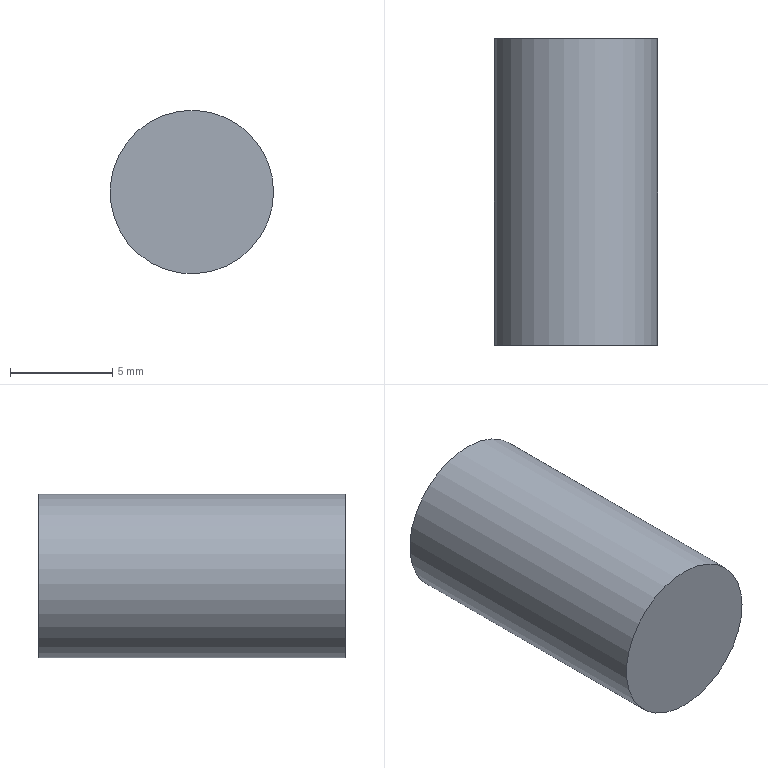Component | NX | 11_SMALL_PISTON | 1 solid | 3 faces | box 8 x 15 x 8 mm | volume 754 mm3 | plane 2 | cylinder 1 | commonest cylinder face diameters 8 x1
STEP:
#1=CARTESIAN_POINT('',(0.,0.,0.));
#2=DIRECTION('',(0.,0.,1.));
#3=DIRECTION('',(1.,0.,0.));
#4=AXIS2_PLACEMENT_3D('',#1,#2,#3);
#5=CARTESIAN_POINT('',(-55.735,168.794,-236.031));
#6=VERTEX_POINT('',#5);
#7=CARTESIAN_POINT('',(-59.084,168.794,-238.219));
#8=DIRECTION('',(0.,-1.,0.));
#9=DIRECTION('',(0.8372,0.,0.5469));
#10=AXIS2_PLACEMENT_3D('',#7,#8,#9);
#11=CIRCLE('',#10,4.);
#12=CARTESIAN_POINT('',(-59.084,168.794,-238.219));
#13=DIRECTION('',(0.,1.,0.));
#14=DIRECTION('',(0.8372,0.,0.5469));
#15=AXIS2_PLACEMENT_3D('',#12,#13,#14);
#16=PLANE('',#15);
#17=CARTESIAN_POINT('',(4.,-0.));
#18=CARTESIAN_POINT('',(4.,-6.928));
#19=CARTESIAN_POINT('',(-2.,-3.464));
#20=CARTESIAN_POINT('',(-8.,0.));
#21=CARTESIAN_POINT('',(-2.,3.464));
#22=CARTESIAN_POINT('',(4.,6.928));
#23=CARTESIAN_POINT('',(4.,-0.));
#24=(BOUNDED_CURVE()B_SPLINE_CURVE(2,(#17,#18,#19,#20,#21,#22,#23),.UNSPECIFIED.,.T.,.F.)B_SPLINE_CURVE_WITH_KNOTS((1,2,2,2,2,1),(-2.094,0.,2.094,4.189,6.283,8.378),.UNSPECIFIED.)CURVE()GEOMETRIC_REPRESENTATION_ITEM()RATIONAL_B_SPLINE_CURVE((1.,0.5,1.,0.5,1.,0.5,1.))REPRESENTATION_ITEM(''));
#25=(GEOMETRIC_REPRESENTATION_CONTEXT(2)PARAMETRIC_REPRESENTATION_CONTEXT()REPRESENTATION_CONTEXT('',''));
#26=DEFINITIONAL_REPRESENTATION('',(#24),#25);
#27=PCURVE('',#16,#26);
#28=CARTESIAN_POINT('',(-59.084,153.794,-238.219));
#29=DIRECTION('',(0.,1.,0.));
#30=DIRECTION('',(0.8372,0.,0.5469));
#31=AXIS2_PLACEMENT_3D('',#28,#29,#30);
#32=CYLINDRICAL_SURFACE('',#31,4.);
#33=CARTESIAN_POINT('',(6.283,15.));
#34=DIRECTION('',(-1.,0.));
#35=VECTOR('',#34,1.);
#36=LINE('',#33,#35);
#37=(GEOMETRIC_REPRESENTATION_CONTEXT(2)PARAMETRIC_REPRESENTATION_CONTEXT()REPRESENTATION_CONTEXT('',''));
#38=DEFINITIONAL_REPRESENTATION('',(#36),#37);
#39=PCURVE('',#32,#38);
#40=SURFACE_CURVE('',#11,(#27,#39),.PCURVE_S1.);
#41=EDGE_CURVE('',#6,#6,#40,.T.);
#42=ORIENTED_EDGE('',*,*,#41,.F.);
#43=EDGE_LOOP('',(#42));
#44=FACE_BOUND('',#43,.T.);
#45=ADVANCED_FACE('',(#44),#16,.T.);
#46=CARTESIAN_POINT('',(-55.735,153.794,-236.031));
#47=VERTEX_POINT('',#46);
#48=CARTESIAN_POINT('',(-59.084,153.794,-238.219));
#49=DIRECTION('',(0.,1.,0.));
#50=DIRECTION('',(0.8372,0.,0.5469));
#51=AXIS2_PLACEMENT_3D('',#48,#49,#50);
#52=CIRCLE('',#51,4.);
#53=CARTESIAN_POINT('',(-59.084,153.794,-238.219));
#54=DIRECTION('',(0.,-1.,0.));
#55=DIRECTION('',(-0.8372,0.,-0.5469));
#56=AXIS2_PLACEMENT_3D('',#53,#54,#55);
#57=PLANE('',#56);
#58=CARTESIAN_POINT('',(-4.,-0.));
#59=CARTESIAN_POINT('',(-4.,6.928));
#60=CARTESIAN_POINT('',(2.,3.464));
#61=CARTESIAN_POINT('',(8.,0.));
#62=CARTESIAN_POINT('',(2.,-3.464));
#63=CARTESIAN_POINT('',(-4.,-6.928));
#64=CARTESIAN_POINT('',(-4.,-0.));
#65=(BOUNDED_CURVE()B_SPLINE_CURVE(2,(#58,#59,#60,#61,#62,#63,#64),.UNSPECIFIED.,.T.,.F.)B_SPLINE_CURVE_WITH_KNOTS((1,2,2,2,2,1),(-2.094,0.,2.094,4.189,6.283,8.378),.UNSPECIFIED.)CURVE()GEOMETRIC_REPRESENTATION_ITEM()RATIONAL_B_SPLINE_CURVE((1.,0.5,1.,0.5,1.,0.5,1.))REPRESENTATION_ITEM(''));
#66=(GEOMETRIC_REPRESENTATION_CONTEXT(2)PARAMETRIC_REPRESENTATION_CONTEXT()REPRESENTATION_CONTEXT('',''));
#67=DEFINITIONAL_REPRESENTATION('',(#65),#66);
#68=PCURVE('',#57,#67);
#69=CARTESIAN_POINT('',(0.,0.));
#70=DIRECTION('',(1.,0.));
#71=VECTOR('',#70,1.);
#72=LINE('',#69,#71);
#73=(GEOMETRIC_REPRESENTATION_CONTEXT(2)PARAMETRIC_REPRESENTATION_CONTEXT()REPRESENTATION_CONTEXT('',''));
#74=DEFINITIONAL_REPRESENTATION('',(#72),#73);
#75=PCURVE('',#32,#74);
#76=SURFACE_CURVE('',#52,(#68,#75),.PCURVE_S1.);
#77=EDGE_CURVE('',#47,#47,#76,.T.);
#78=ORIENTED_EDGE('',*,*,#77,.F.);
#79=EDGE_LOOP('',(#78));
#80=FACE_BOUND('',#79,.T.);
#81=ADVANCED_FACE('',(#80),#57,.T.);
#82=ORIENTED_EDGE('',*,*,#41,.T.);
#83=CARTESIAN_POINT('',(-55.735,153.794,-236.031));
#84=CARTESIAN_POINT('',(-55.735,168.794,-236.031));
#85=B_SPLINE_CURVE_WITH_KNOTS('',1,(#83,#84),.UNSPECIFIED.,.F.,.F.,(2,2),(0.,15.),.PIECEWISE_BEZIER_KNOTS.);
#86=CARTESIAN_POINT('',(0.,0.));
#87=DIRECTION('',(0.,1.));
#88=VECTOR('',#87,1.);
#89=LINE('',#86,#88);
#90=(GEOMETRIC_REPRESENTATION_CONTEXT(2)PARAMETRIC_REPRESENTATION_CONTEXT()REPRESENTATION_CONTEXT('',''));
#91=DEFINITIONAL_REPRESENTATION('',(#89),#90);
#92=PCURVE('',#32,#91);
#93=CARTESIAN_POINT('',(6.283,0.));
#94=DIRECTION('',(0.,1.));
#95=VECTOR('',#94,1.);
#96=LINE('',#93,#95);
#97=(GEOMETRIC_REPRESENTATION_CONTEXT(2)PARAMETRIC_REPRESENTATION_CONTEXT()REPRESENTATION_CONTEXT('',''));
#98=DEFINITIONAL_REPRESENTATION('',(#96),#97);
#99=PCURVE('',#32,#98);
#100=SEAM_CURVE('',#85,(#92,#99),.PCURVE_S1.);
#101=EDGE_CURVE('',#47,#6,#100,.T.);
#102=ORIENTED_EDGE('',*,*,#101,.F.);
#103=ORIENTED_EDGE('',*,*,#77,.T.);
#104=ORIENTED_EDGE('',*,*,#101,.T.);
#105=EDGE_LOOP('',(#82,#102,#103,#104));
#106=FACE_BOUND('',#105,.T.);
#107=ADVANCED_FACE('',(#106),#32,.T.);
#108=CLOSED_SHELL('',(#45,#81,#107));
#109=MANIFOLD_SOLID_BREP('',#108);
#110=(LENGTH_UNIT()NAMED_UNIT(*)SI_UNIT(.MILLI.,.METRE.));
#111=UNCERTAINTY_MEASURE_WITH_UNIT(LENGTH_MEASURE(0.00001),#110,'','');
#112=(NAMED_UNIT(*)PLANE_ANGLE_UNIT()SI_UNIT($,.RADIAN.));
#113=(NAMED_UNIT(*)SI_UNIT($,.STERADIAN.)SOLID_ANGLE_UNIT());
#114=(GEOMETRIC_REPRESENTATION_CONTEXT(3)GLOBAL_UNCERTAINTY_ASSIGNED_CONTEXT((#111))GLOBAL_UNIT_ASSIGNED_CONTEXT((#110,#112,#113))REPRESENTATION_CONTEXT('',''));
#115=ADVANCED_BREP_SHAPE_REPRESENTATION('',(#4,#109),#114);